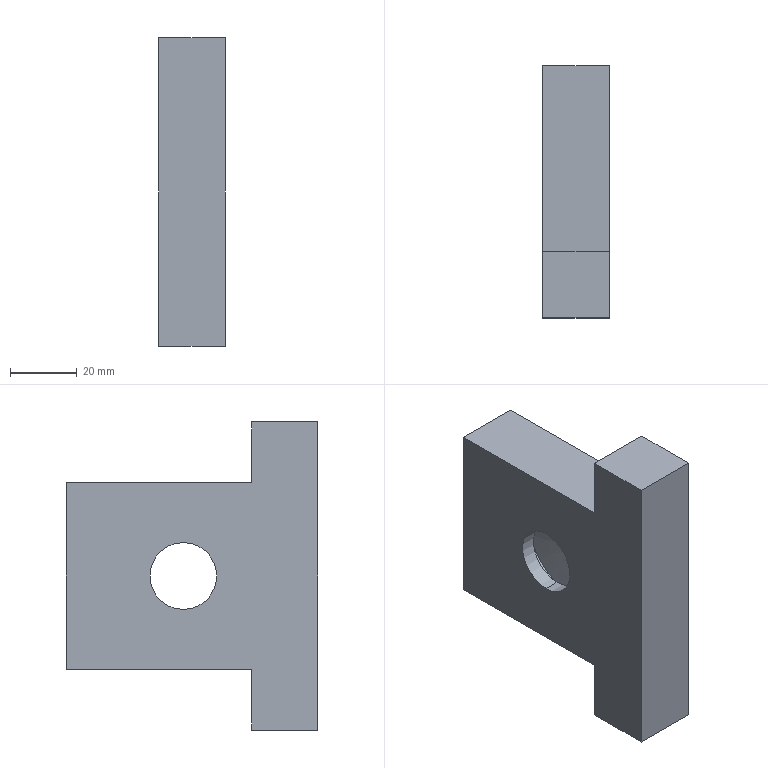Component | SolidWorks | SealingAnvil-1 | 1 solid | 20 faces | box 20 x 75.24 x 92.14 mm | volume 83701 mm3 | plane 10 | cylinder 6 | cone 4 | commonest cylinder face diameters 20 x4 41.575 x2
build123d program:
from build123d import *

# Parameters (mm, degrees)
SKETCH2_R           = 10
BOSS_EXTRUDE1_DEPTH = 20


with BuildPart() as part:
    # Sketch2 → Boss-Extrude1 (new body)
    with BuildSketch(Plane.XY):
        Polygon((27.887, 95.24), (-27.887, 95.24), (-27.887, 39.822), (-46.072, 39.822), (-46.072, 20), (46.072, 20), (46.072, 39.822), (27.887, 39.822), align=None)
        with Locations((0, 60.219)):
            Circle(SKETCH2_R, mode=Mode.SUBTRACT)
    extrude(amount=BOSS_EXTRUDE1_DEPTH)

    # Sketch3 → Cut-Revolve1 (revolve, cut)
    with BuildSketch(Plane(origin=(0, 0, 0), x_dir=(0, 0, -1), z_dir=(1, 0, 0)), mode=Mode.PRIVATE) as cut_revolve1_sk:
        Polygon((-12.9, 81.007), (-15.408, 70.219), (-4.592, 70.219), (-7.1, 81.007), align=None)
    revolve(cut_revolve1_sk.sketch.rotate(Axis((0, 60.219, -248), (0, 0, 1)), 90), axis=Axis((0, 60.219, -248), (0, 0, 1)), mode=Mode.SUBTRACT)


solid = part.part

# Placed as in the assembly
solid = solid.moved(Location((-166, 0, 0), (0, 90, 0)))
STEP:
#1=COLOUR_RGB('',0.7922,0.8196,0.9333);
#2=FILL_AREA_STYLE_COLOUR('',#1);
#3=FILL_AREA_STYLE('',(#2));
#4=SURFACE_STYLE_FILL_AREA(#3);
#5=SURFACE_SIDE_STYLE('',(#4));
#6=SURFACE_STYLE_USAGE(.BOTH.,#5);
#7=PRESENTATION_STYLE_ASSIGNMENT((#6));
#8=CARTESIAN_POINT('',(-6.028,2.371,-0.8184));
#9=VERTEX_POINT('',#8);
#10=CARTESIAN_POINT('',(-6.028,2.371,0.8184));
#11=VERTEX_POINT('',#10);
#12=CARTESIAN_POINT('',(-6.028,2.371,0.));
#13=DIRECTION('',(-1.,0.,0.));
#14=DIRECTION('',(0.,0.,1.));
#15=AXIS2_PLACEMENT_3D('',#12,#13,#14);
#16=CIRCLE('',#15,0.8184);
#17=EDGE_CURVE('',#9,#11,#16,.T.);
#18=ORIENTED_EDGE('',*,*,#17,.F.);
#19=CARTESIAN_POINT('',(-6.256,2.371,-0.8184));
#20=VERTEX_POINT('',#19);
#21=CARTESIAN_POINT('',(-16.299,2.371,-0.8184));
#22=DIRECTION('',(-1.,0.,0.));
#23=VECTOR('',#22,39.37);
#24=LINE('',#21,#23);
#25=EDGE_CURVE('',#9,#20,#24,.T.);
#26=ORIENTED_EDGE('',*,*,#25,.T.);
#27=CARTESIAN_POINT('',(-6.256,2.371,0.8184));
#28=VERTEX_POINT('',#27);
#29=CARTESIAN_POINT('',(-6.256,2.371,0.));
#30=DIRECTION('',(-1.,0.,0.));
#31=DIRECTION('',(0.,0.,1.));
#32=AXIS2_PLACEMENT_3D('',#29,#30,#31);
#33=CIRCLE('',#32,0.8184);
#34=EDGE_CURVE('',#20,#28,#33,.T.);
#35=ORIENTED_EDGE('',*,*,#34,.T.);
#36=CARTESIAN_POINT('',(-16.299,2.371,0.8184));
#37=DIRECTION('',(-1.,0.,0.));
#38=VECTOR('',#37,39.37);
#39=LINE('',#36,#38);
#40=EDGE_CURVE('',#11,#28,#39,.T.);
#41=ORIENTED_EDGE('',*,*,#40,.F.);
#42=EDGE_LOOP('',(#18,#26,#35,#41));
#43=FACE_OUTER_BOUND('',#42,.T.);
#44=CARTESIAN_POINT('',(-16.299,2.371,0.));
#45=DIRECTION('',(-1.,0.,0.));
#46=DIRECTION('',(0.,0.,1.));
#47=AXIS2_PLACEMENT_3D('',#44,#45,#46);
#48=CYLINDRICAL_SURFACE('',#47,0.8184);
#49=ADVANCED_FACE('',(#43),#48,.F.);
#50=CARTESIAN_POINT('',(-6.355,2.371,-0.3937));
#51=VERTEX_POINT('',#50);
#52=CARTESIAN_POINT('',(-6.355,2.371,0.3937));
#53=VERTEX_POINT('',#52);
#54=CARTESIAN_POINT('',(-6.355,2.371,0.));
#55=DIRECTION('',(-1.,0.,0.));
#56=DIRECTION('',(0.,0.,1.));
#57=AXIS2_PLACEMENT_3D('',#54,#55,#56);
#58=CIRCLE('',#57,0.3937);
#59=EDGE_CURVE('',#51,#53,#58,.T.);
#60=ORIENTED_EDGE('',*,*,#59,.T.);
#61=CARTESIAN_POINT('',(-6.355,2.371,0.3937));
#62=DIRECTION('',(0.2264,0.,0.974));
#63=VECTOR('',#62,39.37);
#64=LINE('',#61,#63);
#65=EDGE_CURVE('',#53,#28,#64,.T.);
#66=ORIENTED_EDGE('',*,*,#65,.T.);
#67=ORIENTED_EDGE('',*,*,#34,.F.);
#68=CARTESIAN_POINT('',(-6.355,2.371,-0.3937));
#69=DIRECTION('',(0.2264,0.,-0.974));
#70=VECTOR('',#69,39.37);
#71=LINE('',#68,#70);
#72=EDGE_CURVE('',#51,#20,#71,.T.);
#73=ORIENTED_EDGE('',*,*,#72,.F.);
#74=EDGE_LOOP('',(#60,#66,#67,#73));
#75=FACE_OUTER_BOUND('',#74,.T.);
#76=CARTESIAN_POINT('',(-6.355,2.371,0.));
#77=DIRECTION('',(1.,0.,0.));
#78=DIRECTION('',(0.,0.,-1.));
#79=AXIS2_PLACEMENT_3D('',#76,#77,#78);
#80=CONICAL_SURFACE('',#79,0.3937,1.342);
#81=ADVANCED_FACE('',(#75),#80,.F.);
#82=CARTESIAN_POINT('',(-5.929,2.371,-0.3937));
#83=VERTEX_POINT('',#82);
#84=CARTESIAN_POINT('',(-5.929,2.371,0.3937));
#85=VERTEX_POINT('',#84);
#86=CARTESIAN_POINT('',(-5.929,2.371,0.));
#87=DIRECTION('',(-1.,0.,0.));
#88=DIRECTION('',(0.,0.,1.));
#89=AXIS2_PLACEMENT_3D('',#86,#87,#88);
#90=CIRCLE('',#89,0.3937);
#91=EDGE_CURVE('',#83,#85,#90,.T.);
#92=ORIENTED_EDGE('',*,*,#91,.F.);
#93=CARTESIAN_POINT('',(-5.929,2.371,-0.3937));
#94=DIRECTION('',(-0.2264,0.,-0.974));
#95=VECTOR('',#94,39.37);
#96=LINE('',#93,#95);
#97=EDGE_CURVE('',#83,#9,#96,.T.);
#98=ORIENTED_EDGE('',*,*,#97,.T.);
#99=ORIENTED_EDGE('',*,*,#17,.T.);
#100=CARTESIAN_POINT('',(-5.929,2.371,0.3937));
#101=DIRECTION('',(-0.2264,0.,0.974));
#102=VECTOR('',#101,39.37);
#103=LINE('',#100,#102);
#104=EDGE_CURVE('',#85,#11,#103,.T.);
#105=ORIENTED_EDGE('',*,*,#104,.F.);
#106=EDGE_LOOP('',(#92,#98,#99,#105));
#107=FACE_OUTER_BOUND('',#106,.T.);
#108=CARTESIAN_POINT('',(-5.929,2.371,0.));
#109=DIRECTION('',(-1.,0.,0.));
#110=DIRECTION('',(0.,0.,1.));
#111=AXIS2_PLACEMENT_3D('',#108,#109,#110);
#112=CONICAL_SURFACE('',#111,0.3937,1.342);
#113=ADVANCED_FACE('',(#107),#112,.F.);
#114=ORIENTED_EDGE('',*,*,#59,.F.);
#115=CARTESIAN_POINT('',(-6.535,2.371,-0.3937));
#116=VERTEX_POINT('',#115);
#117=CARTESIAN_POINT('',(-5.748,2.371,-0.3937));
#118=DIRECTION('',(-1.,0.,0.));
#119=VECTOR('',#118,39.37);
#120=LINE('',#117,#119);
#121=EDGE_CURVE('',#51,#116,#120,.T.);
#122=ORIENTED_EDGE('',*,*,#121,.T.);
#123=CARTESIAN_POINT('',(-6.535,2.371,0.3937));
#124=VERTEX_POINT('',#123);
#125=CARTESIAN_POINT('',(-6.535,2.371,-0.));
#126=DIRECTION('',(1.,0.,0.));
#127=DIRECTION('',(0.,0.,-1.));
#128=AXIS2_PLACEMENT_3D('',#125,#126,#127);
#129=CIRCLE('',#128,0.3937);
#130=EDGE_CURVE('',#124,#116,#129,.T.);
#131=ORIENTED_EDGE('',*,*,#130,.F.);
#132=CARTESIAN_POINT('',(-5.748,2.371,0.3937));
#133=DIRECTION('',(-1.,0.,0.));
#134=VECTOR('',#133,39.37);
#135=LINE('',#132,#134);
#136=EDGE_CURVE('',#53,#124,#135,.T.);
#137=ORIENTED_EDGE('',*,*,#136,.F.);
#138=EDGE_LOOP('',(#114,#122,#131,#137));
#139=FACE_OUTER_BOUND('',#138,.T.);
#140=CARTESIAN_POINT('',(-5.748,2.371,-0.));
#141=DIRECTION('',(-1.,0.,0.));
#142=DIRECTION('',(0.,0.,1.));
#143=AXIS2_PLACEMENT_3D('',#140,#141,#142);
#144=CYLINDRICAL_SURFACE('',#143,0.3937);
#145=ADVANCED_FACE('',(#139),#144,.F.);
#146=CARTESIAN_POINT('',(-5.748,2.371,0.3937));
#147=VERTEX_POINT('',#146);
#148=CARTESIAN_POINT('',(-5.748,2.371,-0.3937));
#149=VERTEX_POINT('',#148);
#150=CARTESIAN_POINT('',(-5.748,2.371,-0.));
#151=DIRECTION('',(1.,0.,0.));
#152=DIRECTION('',(0.,0.,-1.));
#153=AXIS2_PLACEMENT_3D('',#150,#151,#152);
#154=CIRCLE('',#153,0.3937);
#155=EDGE_CURVE('',#147,#149,#154,.T.);
#156=ORIENTED_EDGE('',*,*,#155,.T.);
#157=CARTESIAN_POINT('',(-5.748,2.371,-0.3937));
#158=DIRECTION('',(-1.,0.,0.));
#159=VECTOR('',#158,39.37);
#160=LINE('',#157,#159);
#161=EDGE_CURVE('',#149,#83,#160,.T.);
#162=ORIENTED_EDGE('',*,*,#161,.T.);
#163=ORIENTED_EDGE('',*,*,#91,.T.);
#164=CARTESIAN_POINT('',(-5.748,2.371,0.3937));
#165=DIRECTION('',(-1.,0.,0.));
#166=VECTOR('',#165,39.37);
#167=LINE('',#164,#166);
#168=EDGE_CURVE('',#147,#85,#167,.T.);
#169=ORIENTED_EDGE('',*,*,#168,.F.);
#170=EDGE_LOOP('',(#156,#162,#163,#169));
#171=FACE_OUTER_BOUND('',#170,.T.);
#172=CARTESIAN_POINT('',(-5.748,2.371,-0.));
#173=DIRECTION('',(-1.,0.,0.));
#174=DIRECTION('',(0.,0.,1.));
#175=AXIS2_PLACEMENT_3D('',#172,#173,#174);
#176=CYLINDRICAL_SURFACE('',#175,0.3937);
#177=ADVANCED_FACE('',(#171),#176,.F.);
#178=ORIENTED_EDGE('',*,*,#161,.F.);
#179=CARTESIAN_POINT('',(-5.748,2.371,-0.));
#180=DIRECTION('',(1.,0.,0.));
#181=DIRECTION('',(0.,0.,-1.));
#182=AXIS2_PLACEMENT_3D('',#179,#180,#181);
#183=CIRCLE('',#182,0.3937);
#184=EDGE_CURVE('',#149,#147,#183,.T.);
#185=ORIENTED_EDGE('',*,*,#184,.T.);
#186=ORIENTED_EDGE('',*,*,#168,.T.);
#187=CARTESIAN_POINT('',(-5.929,2.371,0.));
#188=DIRECTION('',(-1.,0.,0.));
#189=DIRECTION('',(0.,0.,1.));
#190=AXIS2_PLACEMENT_3D('',#187,#188,#189);
#191=CIRCLE('',#190,0.3937);
#192=EDGE_CURVE('',#85,#83,#191,.T.);
#193=ORIENTED_EDGE('',*,*,#192,.T.);
#194=EDGE_LOOP('',(#178,#185,#186,#193));
#195=FACE_OUTER_BOUND('',#194,.T.);
#196=CARTESIAN_POINT('',(-5.748,2.371,-0.));
#197=DIRECTION('',(-1.,0.,0.));
#198=DIRECTION('',(0.,0.,1.));
#199=AXIS2_PLACEMENT_3D('',#196,#197,#198);
#200=CYLINDRICAL_SURFACE('',#199,0.3937);
#201=ADVANCED_FACE('',(#195),#200,.F.);
#202=CARTESIAN_POINT('',(-5.748,1.568,-1.098));
#203=VERTEX_POINT('',#202);
#204=CARTESIAN_POINT('',(-5.748,3.75,-1.098));
#205=VERTEX_POINT('',#204);
#206=CARTESIAN_POINT('',(-5.748,1.568,-1.098));
#207=DIRECTION('',(0.,1.,0.));
#208=VECTOR('',#207,39.37);
#209=LINE('',#206,#208);
#210=EDGE_CURVE('',#203,#205,#209,.T.);
#211=ORIENTED_EDGE('',*,*,#210,.T.);
#212=CARTESIAN_POINT('',(-5.748,3.75,1.098));
#213=VERTEX_POINT('',#212);
#214=CARTESIAN_POINT('',(-5.748,3.75,-1.098));
#215=DIRECTION('',(0.,0.,1.));
#216=VECTOR('',#215,39.37);
#217=LINE('',#214,#216);
#218=EDGE_CURVE('',#205,#213,#217,.T.);
#219=ORIENTED_EDGE('',*,*,#218,.T.);
#220=CARTESIAN_POINT('',(-5.748,1.568,1.098));
#221=VERTEX_POINT('',#220);
#222=CARTESIAN_POINT('',(-5.748,3.75,1.098));
#223=DIRECTION('',(0.,-1.,0.));
#224=VECTOR('',#223,39.37);
#225=LINE('',#222,#224);
#226=EDGE_CURVE('',#213,#221,#225,.T.);
#227=ORIENTED_EDGE('',*,*,#226,.T.);
#228=CARTESIAN_POINT('',(-5.748,1.568,1.814));
#229=VERTEX_POINT('',#228);
#230=CARTESIAN_POINT('',(-5.748,1.568,1.098));
#231=DIRECTION('',(0.,-0.,1.));
#232=VECTOR('',#231,39.37);
#233=LINE('',#230,#232);
#234=EDGE_CURVE('',#221,#229,#233,.T.);
#235=ORIENTED_EDGE('',*,*,#234,.T.);
#236=CARTESIAN_POINT('',(-5.748,0.7874,1.814));
#237=VERTEX_POINT('',#236);
#238=CARTESIAN_POINT('',(-5.748,1.568,1.814));
#239=DIRECTION('',(0.,-1.,-0.));
#240=VECTOR('',#239,39.37);
#241=LINE('',#238,#240);
#242=EDGE_CURVE('',#229,#237,#241,.T.);
#243=ORIENTED_EDGE('',*,*,#242,.T.);
#244=CARTESIAN_POINT('',(-5.748,0.7874,-1.814));
#245=VERTEX_POINT('',#244);
#246=CARTESIAN_POINT('',(-5.748,0.7874,1.814));
#247=DIRECTION('',(0.,0.,-1.));
#248=VECTOR('',#247,39.37);
#249=LINE('',#246,#248);
#250=EDGE_CURVE('',#237,#245,#249,.T.);
#251=ORIENTED_EDGE('',*,*,#250,.T.);
#252=CARTESIAN_POINT('',(-5.748,1.568,-1.814));
#253=VERTEX_POINT('',#252);
#254=CARTESIAN_POINT('',(-5.748,0.7874,-1.814));
#255=DIRECTION('',(0.,1.,0.));
#256=VECTOR('',#255,39.37);
#257=LINE('',#254,#256);
#258=EDGE_CURVE('',#245,#253,#257,.T.);
#259=ORIENTED_EDGE('',*,*,#258,.T.);
#260=CARTESIAN_POINT('',(-5.748,1.568,-1.814));
#261=DIRECTION('',(0.,0.,1.));
#262=VECTOR('',#261,39.37);
#263=LINE('',#260,#262);
#264=EDGE_CURVE('',#253,#203,#263,.T.);
#265=ORIENTED_EDGE('',*,*,#264,.T.);
#266=EDGE_LOOP('',(#211,#219,#227,#235,#243,#251,#259,#265));
#267=FACE_OUTER_BOUND('',#266,.T.);
#268=ORIENTED_EDGE('',*,*,#155,.F.);
#269=ORIENTED_EDGE('',*,*,#184,.F.);
#270=EDGE_LOOP('',(#268,#269));
#271=FACE_BOUND('',#270,.T.);
#272=CARTESIAN_POINT('',(-5.748,-0.,0.));
#273=DIRECTION('',(1.,0.,0.));
#274=DIRECTION('',(0.,0.,-1.));
#275=AXIS2_PLACEMENT_3D('',#272,#273,#274);
#276=PLANE('',#275);
#277=ADVANCED_FACE('',(#267,#271),#276,.T.);
#278=CARTESIAN_POINT('',(-6.535,1.568,-1.098));
#279=VERTEX_POINT('',#278);
#280=CARTESIAN_POINT('',(-6.535,3.75,-1.098));
#281=VERTEX_POINT('',#280);
#282=CARTESIAN_POINT('',(-6.535,1.568,-1.098));
#283=DIRECTION('',(0.,1.,0.));
#284=VECTOR('',#283,39.37);
#285=LINE('',#282,#284);
#286=EDGE_CURVE('',#279,#281,#285,.T.);
#287=ORIENTED_EDGE('',*,*,#286,.F.);
#288=CARTESIAN_POINT('',(-6.535,1.568,-1.814));
#289=VERTEX_POINT('',#288);
#290=CARTESIAN_POINT('',(-6.535,1.568,-1.814));
#291=DIRECTION('',(0.,0.,1.));
#292=VECTOR('',#291,39.37);
#293=LINE('',#290,#292);
#294=EDGE_CURVE('',#289,#279,#293,.T.);
#295=ORIENTED_EDGE('',*,*,#294,.F.);
#296=CARTESIAN_POINT('',(-6.535,0.7874,-1.814));
#297=VERTEX_POINT('',#296);
#298=CARTESIAN_POINT('',(-6.535,0.7874,-1.814));
#299=DIRECTION('',(0.,1.,0.));
#300=VECTOR('',#299,39.37);
#301=LINE('',#298,#300);
#302=EDGE_CURVE('',#297,#289,#301,.T.);
#303=ORIENTED_EDGE('',*,*,#302,.F.);
#304=CARTESIAN_POINT('',(-6.535,0.7874,1.814));
#305=VERTEX_POINT('',#304);
#306=CARTESIAN_POINT('',(-6.535,0.7874,1.814));
#307=DIRECTION('',(0.,0.,-1.));
#308=VECTOR('',#307,39.37);
#309=LINE('',#306,#308);
#310=EDGE_CURVE('',#305,#297,#309,.T.);
#311=ORIENTED_EDGE('',*,*,#310,.F.);
#312=CARTESIAN_POINT('',(-6.535,1.568,1.814));
#313=VERTEX_POINT('',#312);
#314=CARTESIAN_POINT('',(-6.535,1.568,1.814));
#315=DIRECTION('',(0.,-1.,-0.));
#316=VECTOR('',#315,39.37);
#317=LINE('',#314,#316);
#318=EDGE_CURVE('',#313,#305,#317,.T.);
#319=ORIENTED_EDGE('',*,*,#318,.F.);
#320=CARTESIAN_POINT('',(-6.535,1.568,1.098));
#321=VERTEX_POINT('',#320);
#322=CARTESIAN_POINT('',(-6.535,1.568,1.098));
#323=DIRECTION('',(0.,-0.,1.));
#324=VECTOR('',#323,39.37);
#325=LINE('',#322,#324);
#326=EDGE_CURVE('',#321,#313,#325,.T.);
#327=ORIENTED_EDGE('',*,*,#326,.F.);
#328=CARTESIAN_POINT('',(-6.535,3.75,1.098));
#329=VERTEX_POINT('',#328);
#330=CARTESIAN_POINT('',(-6.535,3.75,1.098));
#331=DIRECTION('',(0.,-1.,0.));
#332=VECTOR('',#331,39.37);
#333=LINE('',#330,#332);
#334=EDGE_CURVE('',#329,#321,#333,.T.);
#335=ORIENTED_EDGE('',*,*,#334,.F.);
#336=CARTESIAN_POINT('',(-6.535,3.75,-1.098));
#337=DIRECTION('',(0.,0.,1.));
#338=VECTOR('',#337,39.37);
#339=LINE('',#336,#338);
#340=EDGE_CURVE('',#281,#329,#339,.T.);
#341=ORIENTED_EDGE('',*,*,#340,.F.);
#342=EDGE_LOOP('',(#287,#295,#303,#311,#319,#327,#335,#341));
#343=FACE_OUTER_BOUND('',#342,.T.);
#344=ORIENTED_EDGE('',*,*,#130,.T.);
#345=CARTESIAN_POINT('',(-6.535,2.371,-0.));
#346=DIRECTION('',(1.,0.,0.));
#347=DIRECTION('',(0.,0.,-1.));
#348=AXIS2_PLACEMENT_3D('',#345,#346,#347);
#349=CIRCLE('',#348,0.3937);
#350=EDGE_CURVE('',#116,#124,#349,.T.);
#351=ORIENTED_EDGE('',*,*,#350,.T.);
#352=EDGE_LOOP('',(#344,#351));
#353=FACE_BOUND('',#352,.T.);
#354=CARTESIAN_POINT('',(-6.535,-0.,0.));
#355=DIRECTION('',(1.,0.,0.));
#356=DIRECTION('',(0.,0.,-1.));
#357=AXIS2_PLACEMENT_3D('',#354,#355,#356);
#358=PLANE('',#357);
#359=ADVANCED_FACE('',(#343,#353),#358,.F.);
#360=ORIENTED_EDGE('',*,*,#286,.T.);
#361=CARTESIAN_POINT('',(-5.748,3.75,-1.098));
#362=DIRECTION('',(-1.,0.,0.));
#363=VECTOR('',#362,39.37);
#364=LINE('',#361,#363);
#365=EDGE_CURVE('',#205,#281,#364,.T.);
#366=ORIENTED_EDGE('',*,*,#365,.F.);
#367=ORIENTED_EDGE('',*,*,#210,.F.);
#368=CARTESIAN_POINT('',(-5.748,1.568,-1.098));
#369=DIRECTION('',(-1.,0.,0.));
#370=VECTOR('',#369,39.37);
#371=LINE('',#368,#370);
#372=EDGE_CURVE('',#203,#279,#371,.T.);
#373=ORIENTED_EDGE('',*,*,#372,.T.);
#374=EDGE_LOOP('',(#360,#366,#367,#373));
#375=FACE_OUTER_BOUND('',#374,.T.);
#376=CARTESIAN_POINT('',(-5.748,1.568,-1.098));
#377=DIRECTION('',(0.,0.,1.));
#378=DIRECTION('',(1.,0.,0.));
#379=AXIS2_PLACEMENT_3D('',#376,#377,#378);
#380=PLANE('',#379);
#381=ADVANCED_FACE('',(#375),#380,.F.);
#382=ORIENTED_EDGE('',*,*,#340,.T.);
#383=CARTESIAN_POINT('',(-5.748,3.75,1.098));
#384=DIRECTION('',(-1.,0.,0.));
#385=VECTOR('',#384,39.37);
#386=LINE('',#383,#385);
#387=EDGE_CURVE('',#213,#329,#386,.T.);
#388=ORIENTED_EDGE('',*,*,#387,.F.);
#389=ORIENTED_EDGE('',*,*,#218,.F.);
#390=ORIENTED_EDGE('',*,*,#365,.T.);
#391=EDGE_LOOP('',(#382,#388,#389,#390));
#392=FACE_OUTER_BOUND('',#391,.T.);
#393=CARTESIAN_POINT('',(-5.748,3.75,-1.098));
#394=DIRECTION('',(0.,-1.,0.));
#395=DIRECTION('',(-1.,0.,0.));
#396=AXIS2_PLACEMENT_3D('',#393,#394,#395);
#397=PLANE('',#396);
#398=ADVANCED_FACE('',(#392),#397,.F.);
#399=ORIENTED_EDGE('',*,*,#334,.T.);
#400=CARTESIAN_POINT('',(-5.748,1.568,1.098));
#401=DIRECTION('',(-1.,0.,0.));
#402=VECTOR('',#401,39.37);
#403=LINE('',#400,#402);
#404=EDGE_CURVE('',#221,#321,#403,.T.);
#405=ORIENTED_EDGE('',*,*,#404,.F.);
#406=ORIENTED_EDGE('',*,*,#226,.F.);
#407=ORIENTED_EDGE('',*,*,#387,.T.);
#408=EDGE_LOOP('',(#399,#405,#406,#407));
#409=FACE_OUTER_BOUND('',#408,.T.);
#410=CARTESIAN_POINT('',(-5.748,3.75,1.098));
#411=DIRECTION('',(0.,0.,-1.));
#412=DIRECTION('',(-1.,0.,0.));
#413=AXIS2_PLACEMENT_3D('',#410,#411,#412);
#414=PLANE('',#413);
#415=ADVANCED_FACE('',(#409),#414,.F.);
#416=ORIENTED_EDGE('',*,*,#326,.T.);
#417=CARTESIAN_POINT('',(-5.748,1.568,1.814));
#418=DIRECTION('',(-1.,0.,0.));
#419=VECTOR('',#418,39.37);
#420=LINE('',#417,#419);
#421=EDGE_CURVE('',#229,#313,#420,.T.);
#422=ORIENTED_EDGE('',*,*,#421,.F.);
#423=ORIENTED_EDGE('',*,*,#234,.F.);
#424=ORIENTED_EDGE('',*,*,#404,.T.);
#425=EDGE_LOOP('',(#416,#422,#423,#424));
#426=FACE_OUTER_BOUND('',#425,.T.);
#427=CARTESIAN_POINT('',(-5.748,1.568,1.098));
#428=DIRECTION('',(0.,-1.,-0.));
#429=DIRECTION('',(0.,0.,-1.));
#430=AXIS2_PLACEMENT_3D('',#427,#428,#429);
#431=PLANE('',#430);
#432=ADVANCED_FACE('',(#426),#431,.F.);
#433=ORIENTED_EDGE('',*,*,#318,.T.);
#434=CARTESIAN_POINT('',(-5.748,0.7874,1.814));
#435=DIRECTION('',(-1.,0.,0.));
#436=VECTOR('',#435,39.37);
#437=LINE('',#434,#436);
#438=EDGE_CURVE('',#237,#305,#437,.T.);
#439=ORIENTED_EDGE('',*,*,#438,.F.);
#440=ORIENTED_EDGE('',*,*,#242,.F.);
#441=ORIENTED_EDGE('',*,*,#421,.T.);
#442=EDGE_LOOP('',(#433,#439,#440,#441));
#443=FACE_OUTER_BOUND('',#442,.T.);
#444=CARTESIAN_POINT('',(-5.748,1.568,1.814));
#445=DIRECTION('',(0.,0.,-1.));
#446=DIRECTION('',(0.,1.,0.));
#447=AXIS2_PLACEMENT_3D('',#444,#445,#446);
#448=PLANE('',#447);
#449=ADVANCED_FACE('',(#443),#448,.F.);
#450=ORIENTED_EDGE('',*,*,#310,.T.);
#451=CARTESIAN_POINT('',(-5.748,0.7874,-1.814));
#452=DIRECTION('',(-1.,0.,0.));
#453=VECTOR('',#452,39.37);
#454=LINE('',#451,#453);
#455=EDGE_CURVE('',#245,#297,#454,.T.);
#456=ORIENTED_EDGE('',*,*,#455,.F.);
#457=ORIENTED_EDGE('',*,*,#250,.F.);
#458=ORIENTED_EDGE('',*,*,#438,.T.);
#459=EDGE_LOOP('',(#450,#456,#457,#458));
#460=FACE_OUTER_BOUND('',#459,.T.);
#461=CARTESIAN_POINT('',(-5.748,0.7874,1.814));
#462=DIRECTION('',(0.,1.,0.));
#463=DIRECTION('',(0.,-0.,1.));
#464=AXIS2_PLACEMENT_3D('',#461,#462,#463);
#465=PLANE('',#464);
#466=ADVANCED_FACE('',(#460),#465,.F.);
#467=ORIENTED_EDGE('',*,*,#302,.T.);
#468=CARTESIAN_POINT('',(-5.748,1.568,-1.814));
#469=DIRECTION('',(-1.,0.,0.));
#470=VECTOR('',#469,39.37);
#471=LINE('',#468,#470);
#472=EDGE_CURVE('',#253,#289,#471,.T.);
#473=ORIENTED_EDGE('',*,*,#472,.F.);
#474=ORIENTED_EDGE('',*,*,#258,.F.);
#475=ORIENTED_EDGE('',*,*,#455,.T.);
#476=EDGE_LOOP('',(#467,#473,#474,#475));
#477=FACE_OUTER_BOUND('',#476,.T.);
#478=CARTESIAN_POINT('',(-5.748,0.7874,-1.814));
#479=DIRECTION('',(0.,0.,1.));
#480=DIRECTION('',(1.,0.,0.));
#481=AXIS2_PLACEMENT_3D('',#478,#479,#480);
#482=PLANE('',#481);
#483=ADVANCED_FACE('',(#477),#482,.F.);
#484=ORIENTED_EDGE('',*,*,#294,.T.);
#485=ORIENTED_EDGE('',*,*,#372,.F.);
#486=ORIENTED_EDGE('',*,*,#264,.F.);
#487=ORIENTED_EDGE('',*,*,#472,.T.);
#488=EDGE_LOOP('',(#484,#485,#486,#487));
#489=FACE_OUTER_BOUND('',#488,.T.);
#490=CARTESIAN_POINT('',(-5.748,1.568,-1.814));
#491=DIRECTION('',(0.,-1.,0.));
#492=DIRECTION('',(-1.,0.,0.));
#493=AXIS2_PLACEMENT_3D('',#490,#491,#492);
#494=PLANE('',#493);
#495=ADVANCED_FACE('',(#489),#494,.F.);
#496=ORIENTED_EDGE('',*,*,#121,.F.);
#497=CARTESIAN_POINT('',(-6.355,2.371,0.));
#498=DIRECTION('',(-1.,0.,0.));
#499=DIRECTION('',(0.,0.,1.));
#500=AXIS2_PLACEMENT_3D('',#497,#498,#499);
#501=CIRCLE('',#500,0.3937);
#502=EDGE_CURVE('',#53,#51,#501,.T.);
#503=ORIENTED_EDGE('',*,*,#502,.F.);
#504=ORIENTED_EDGE('',*,*,#136,.T.);
#505=ORIENTED_EDGE('',*,*,#350,.F.);
#506=EDGE_LOOP('',(#496,#503,#504,#505));
#507=FACE_OUTER_BOUND('',#506,.T.);
#508=CARTESIAN_POINT('',(-5.748,2.371,-0.));
#509=DIRECTION('',(-1.,0.,0.));
#510=DIRECTION('',(0.,0.,1.));
#511=AXIS2_PLACEMENT_3D('',#508,#509,#510);
#512=CYLINDRICAL_SURFACE('',#511,0.3937);
#513=ADVANCED_FACE('',(#507),#512,.F.);
#514=ORIENTED_EDGE('',*,*,#97,.F.);
#515=ORIENTED_EDGE('',*,*,#192,.F.);
#516=ORIENTED_EDGE('',*,*,#104,.T.);
#517=CARTESIAN_POINT('',(-6.028,2.371,0.));
#518=DIRECTION('',(-1.,0.,0.));
#519=DIRECTION('',(0.,0.,1.));
#520=AXIS2_PLACEMENT_3D('',#517,#518,#519);
#521=CIRCLE('',#520,0.8184);
#522=EDGE_CURVE('',#11,#9,#521,.T.);
#523=ORIENTED_EDGE('',*,*,#522,.T.);
#524=EDGE_LOOP('',(#514,#515,#516,#523));
#525=FACE_OUTER_BOUND('',#524,.T.);
#526=CARTESIAN_POINT('',(-5.929,2.371,0.));
#527=DIRECTION('',(-1.,0.,0.));
#528=DIRECTION('',(0.,0.,1.));
#529=AXIS2_PLACEMENT_3D('',#526,#527,#528);
#530=CONICAL_SURFACE('',#529,0.3937,1.342);
#531=ADVANCED_FACE('',(#525),#530,.F.);
#532=ORIENTED_EDGE('',*,*,#65,.F.);
#533=ORIENTED_EDGE('',*,*,#502,.T.);
#534=ORIENTED_EDGE('',*,*,#72,.T.);
#535=CARTESIAN_POINT('',(-6.256,2.371,0.));
#536=DIRECTION('',(-1.,0.,0.));
#537=DIRECTION('',(0.,0.,1.));
#538=AXIS2_PLACEMENT_3D('',#535,#536,#537);
#539=CIRCLE('',#538,0.8184);
#540=EDGE_CURVE('',#28,#20,#539,.T.);
#541=ORIENTED_EDGE('',*,*,#540,.F.);
#542=EDGE_LOOP('',(#532,#533,#534,#541));
#543=FACE_OUTER_BOUND('',#542,.T.);
#544=CARTESIAN_POINT('',(-6.355,2.371,0.));
#545=DIRECTION('',(1.,0.,0.));
#546=DIRECTION('',(0.,0.,-1.));
#547=AXIS2_PLACEMENT_3D('',#544,#545,#546);
#548=CONICAL_SURFACE('',#547,0.3937,1.342);
#549=ADVANCED_FACE('',(#543),#548,.F.);
#550=ORIENTED_EDGE('',*,*,#25,.F.);
#551=ORIENTED_EDGE('',*,*,#522,.F.);
#552=ORIENTED_EDGE('',*,*,#40,.T.);
#553=ORIENTED_EDGE('',*,*,#540,.T.);
#554=EDGE_LOOP('',(#550,#551,#552,#553));
#555=FACE_OUTER_BOUND('',#554,.T.);
#556=CARTESIAN_POINT('',(-16.299,2.371,0.));
#557=DIRECTION('',(-1.,0.,0.));
#558=DIRECTION('',(0.,0.,1.));
#559=AXIS2_PLACEMENT_3D('',#556,#557,#558);
#560=CYLINDRICAL_SURFACE('',#559,0.8184);
#561=ADVANCED_FACE('',(#555),#560,.F.);
#562=CLOSED_SHELL('',(#49,#81,#113,#145,#177,#201,#277,#359,#381,#398,#415,#432,#449,#466,#483,#495,#513,#531,#549,#561));
#563=MANIFOLD_SOLID_BREP('',#562);
#564=STYLED_ITEM('',(#7),#563);
#565=(LENGTH_UNIT()NAMED_UNIT(*)SI_UNIT($,.METRE.));
#566=LENGTH_MEASURE_WITH_UNIT(LENGTH_MEASURE(0.0254),#565);
#567=DIMENSIONAL_EXPONENTS(1.,0.,0.,0.,0.,0.,0.);
#568=(CONVERSION_BASED_UNIT('',#566)LENGTH_UNIT()NAMED_UNIT(#567));
#569=UNCERTAINTY_MEASURE_WITH_UNIT(LENGTH_MEASURE(0.00001),#568,'','');
#570=(NAMED_UNIT(*)PLANE_ANGLE_UNIT()SI_UNIT($,.RADIAN.));
#571=(NAMED_UNIT(*)SI_UNIT($,.STERADIAN.)SOLID_ANGLE_UNIT());
#572=(GEOMETRIC_REPRESENTATION_CONTEXT(3)GLOBAL_UNCERTAINTY_ASSIGNED_CONTEXT((#569))GLOBAL_UNIT_ASSIGNED_CONTEXT((#568,#570,#571))REPRESENTATION_CONTEXT('',''));
#573=MECHANICAL_DESIGN_GEOMETRIC_PRESENTATION_REPRESENTATION('',(#564),#572);
#574=CARTESIAN_POINT('',(0.,0.,0.));
#575=DIRECTION('',(0.,0.,1.));
#576=DIRECTION('',(1.,0.,0.));
#577=AXIS2_PLACEMENT_3D('',#574,#575,#576);
#578=(LENGTH_UNIT()NAMED_UNIT(*)SI_UNIT($,.METRE.));
#579=LENGTH_MEASURE_WITH_UNIT(LENGTH_MEASURE(0.0254),#578);
#580=DIMENSIONAL_EXPONENTS(1.,0.,0.,0.,0.,0.,0.);
#581=(CONVERSION_BASED_UNIT('',#579)LENGTH_UNIT()NAMED_UNIT(#580));
#582=UNCERTAINTY_MEASURE_WITH_UNIT(LENGTH_MEASURE(0.00001),#581,'','');
#583=(NAMED_UNIT(*)PLANE_ANGLE_UNIT()SI_UNIT($,.RADIAN.));
#584=(NAMED_UNIT(*)SI_UNIT($,.STERADIAN.)SOLID_ANGLE_UNIT());
#585=(GEOMETRIC_REPRESENTATION_CONTEXT(3)GLOBAL_UNCERTAINTY_ASSIGNED_CONTEXT((#582))GLOBAL_UNIT_ASSIGNED_CONTEXT((#581,#583,#584))REPRESENTATION_CONTEXT('',''));
#586=ADVANCED_BREP_SHAPE_REPRESENTATION('',(#563,#577),#585);
#587=PRESENTATION_LAYER_ASSIGNMENT('','',(#564));